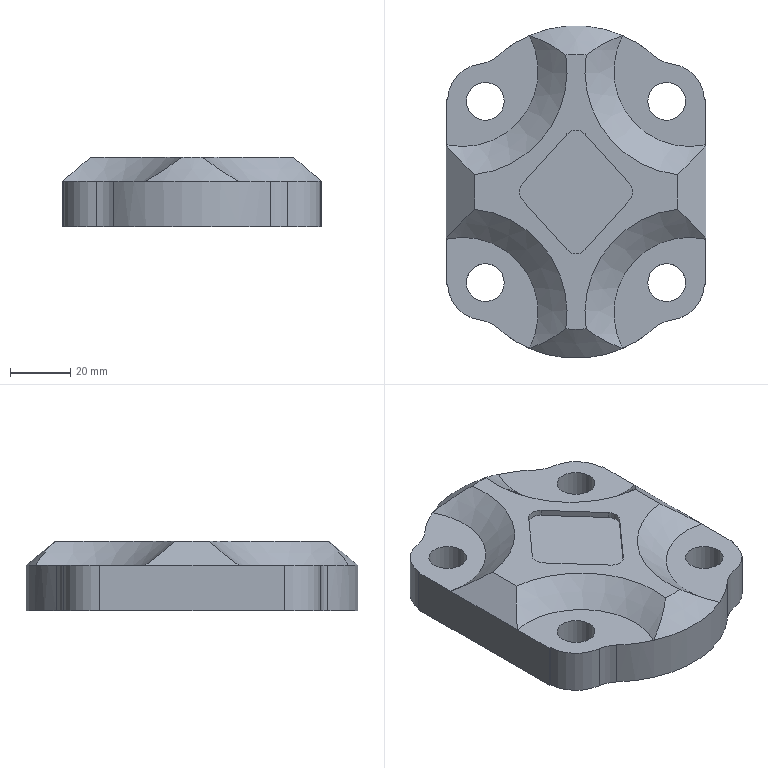Component | NX | 6 | 1 solid | 47 faces | volume 137585 mm3 | plane 21 | cylinder 20 | cone 6 | commonest cylinder face diameters 25 x4 20 x4 12.5 x4 8 x4 77 x2 15 x2